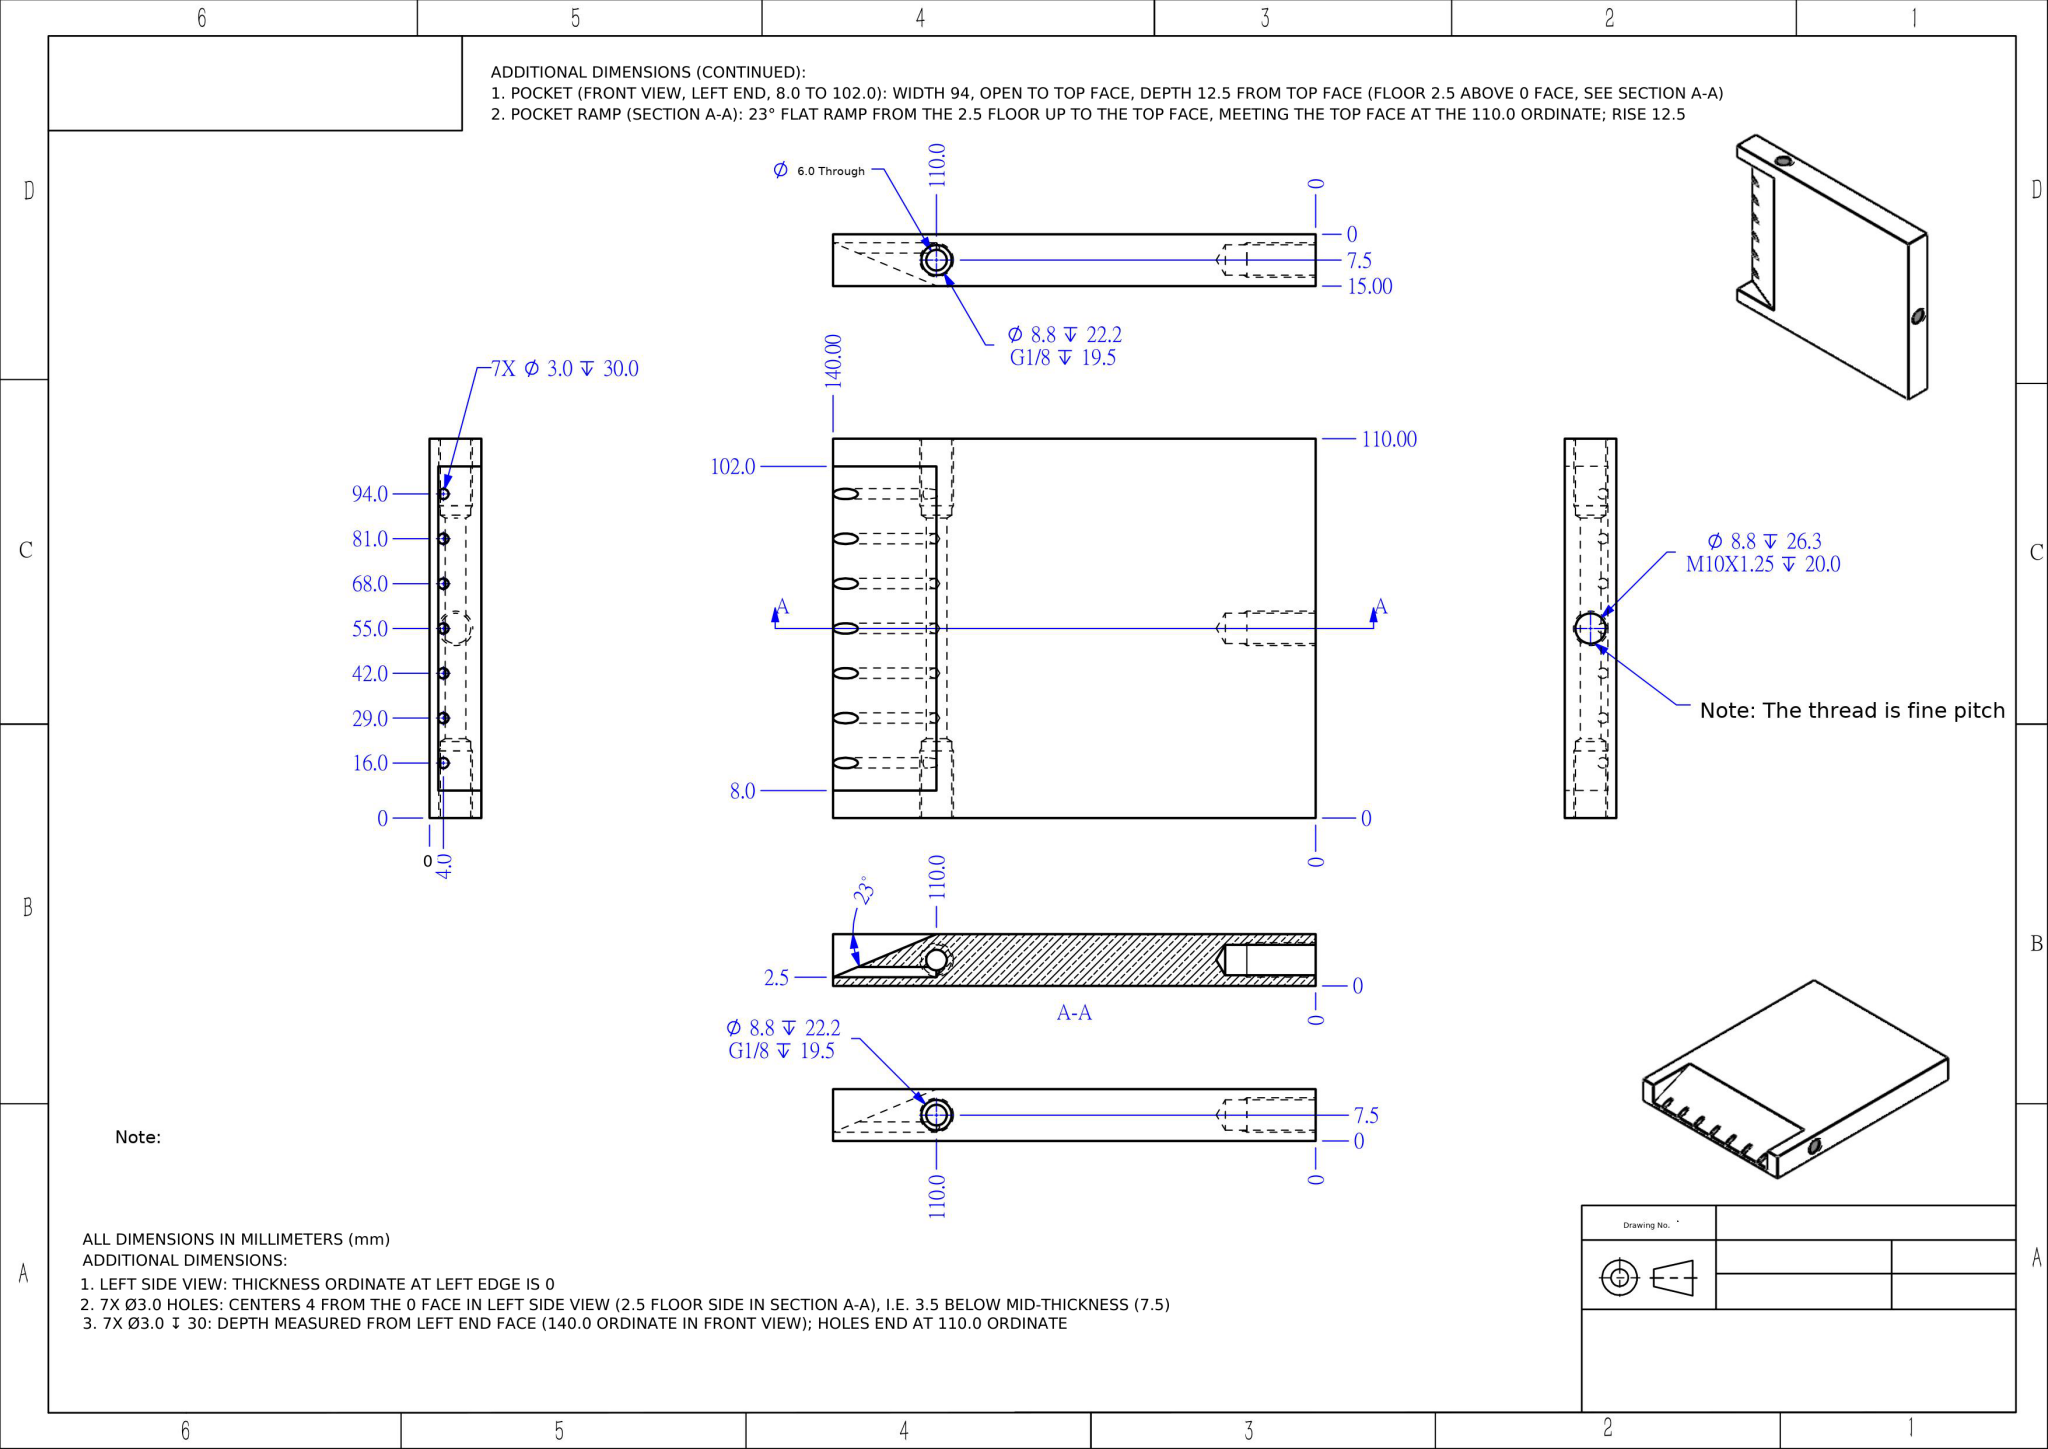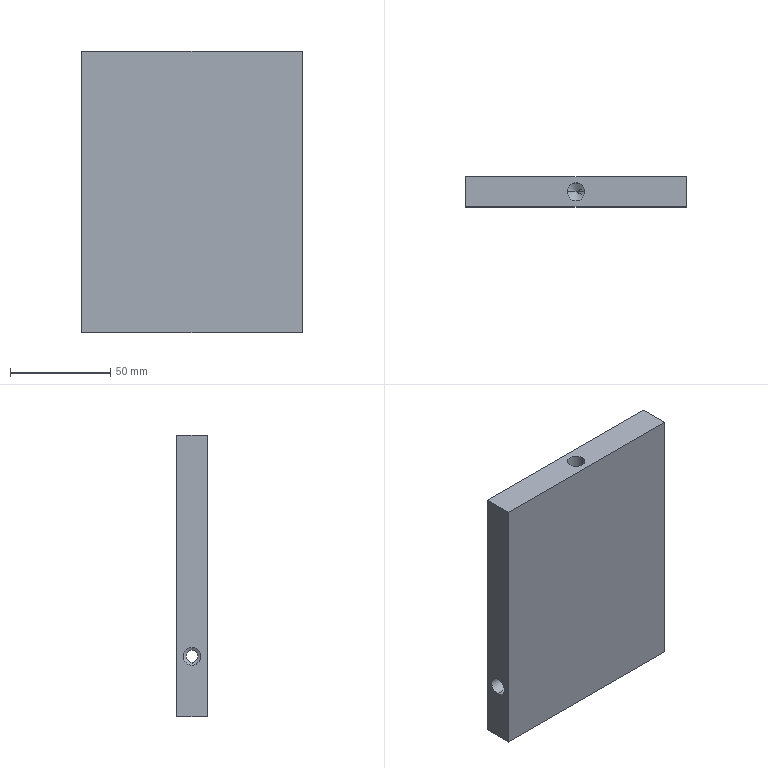Part | NX | mm | 1 solid | 49 faces | box 110 x 15 x 140 mm | volume 205878 mm3 | cylinder 22 | cone 18 | plane 9 | commonest cylinder face diameters 3 x14 8.8 x6 6 x2